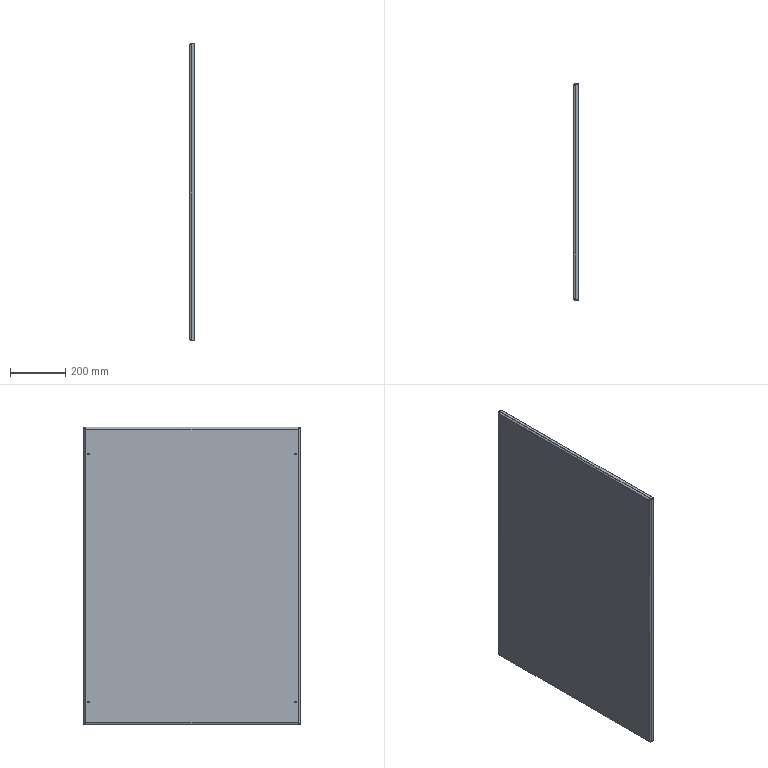Component | SolidWorks | RearUpperDoorPanel(No.27)-1 | 1 solid | 46 faces | volume 1792613 mm3 | plane 22 | cylinder 16 | spline 8 | commonest cylinder face diameters 6.5 x8 14 x4 10 x4 | material Plain Carbon Steel